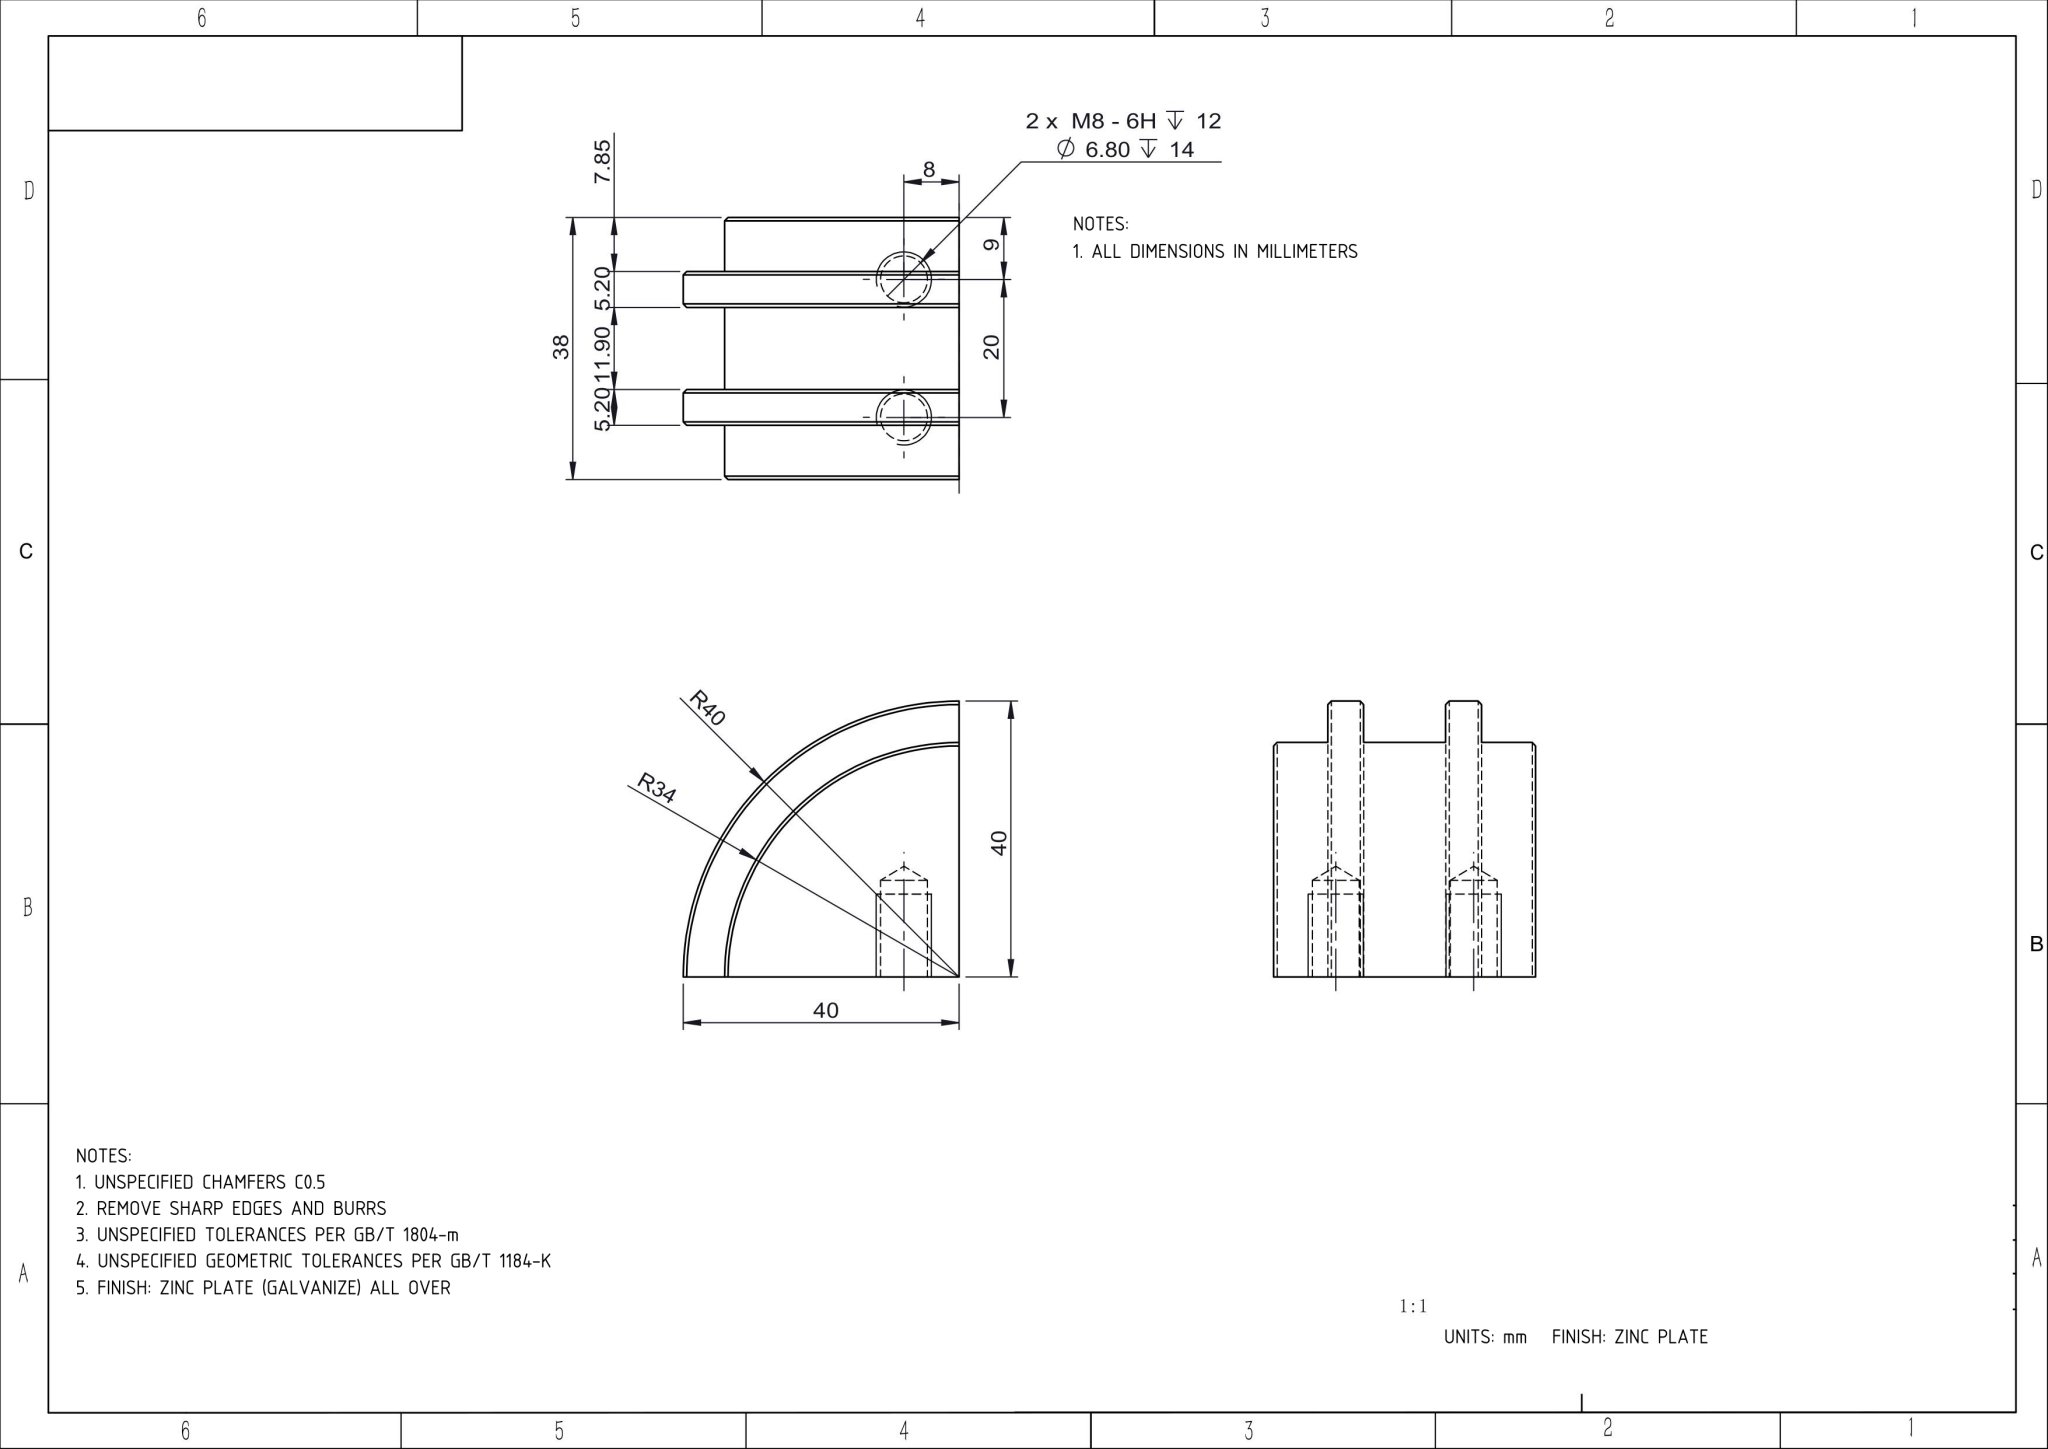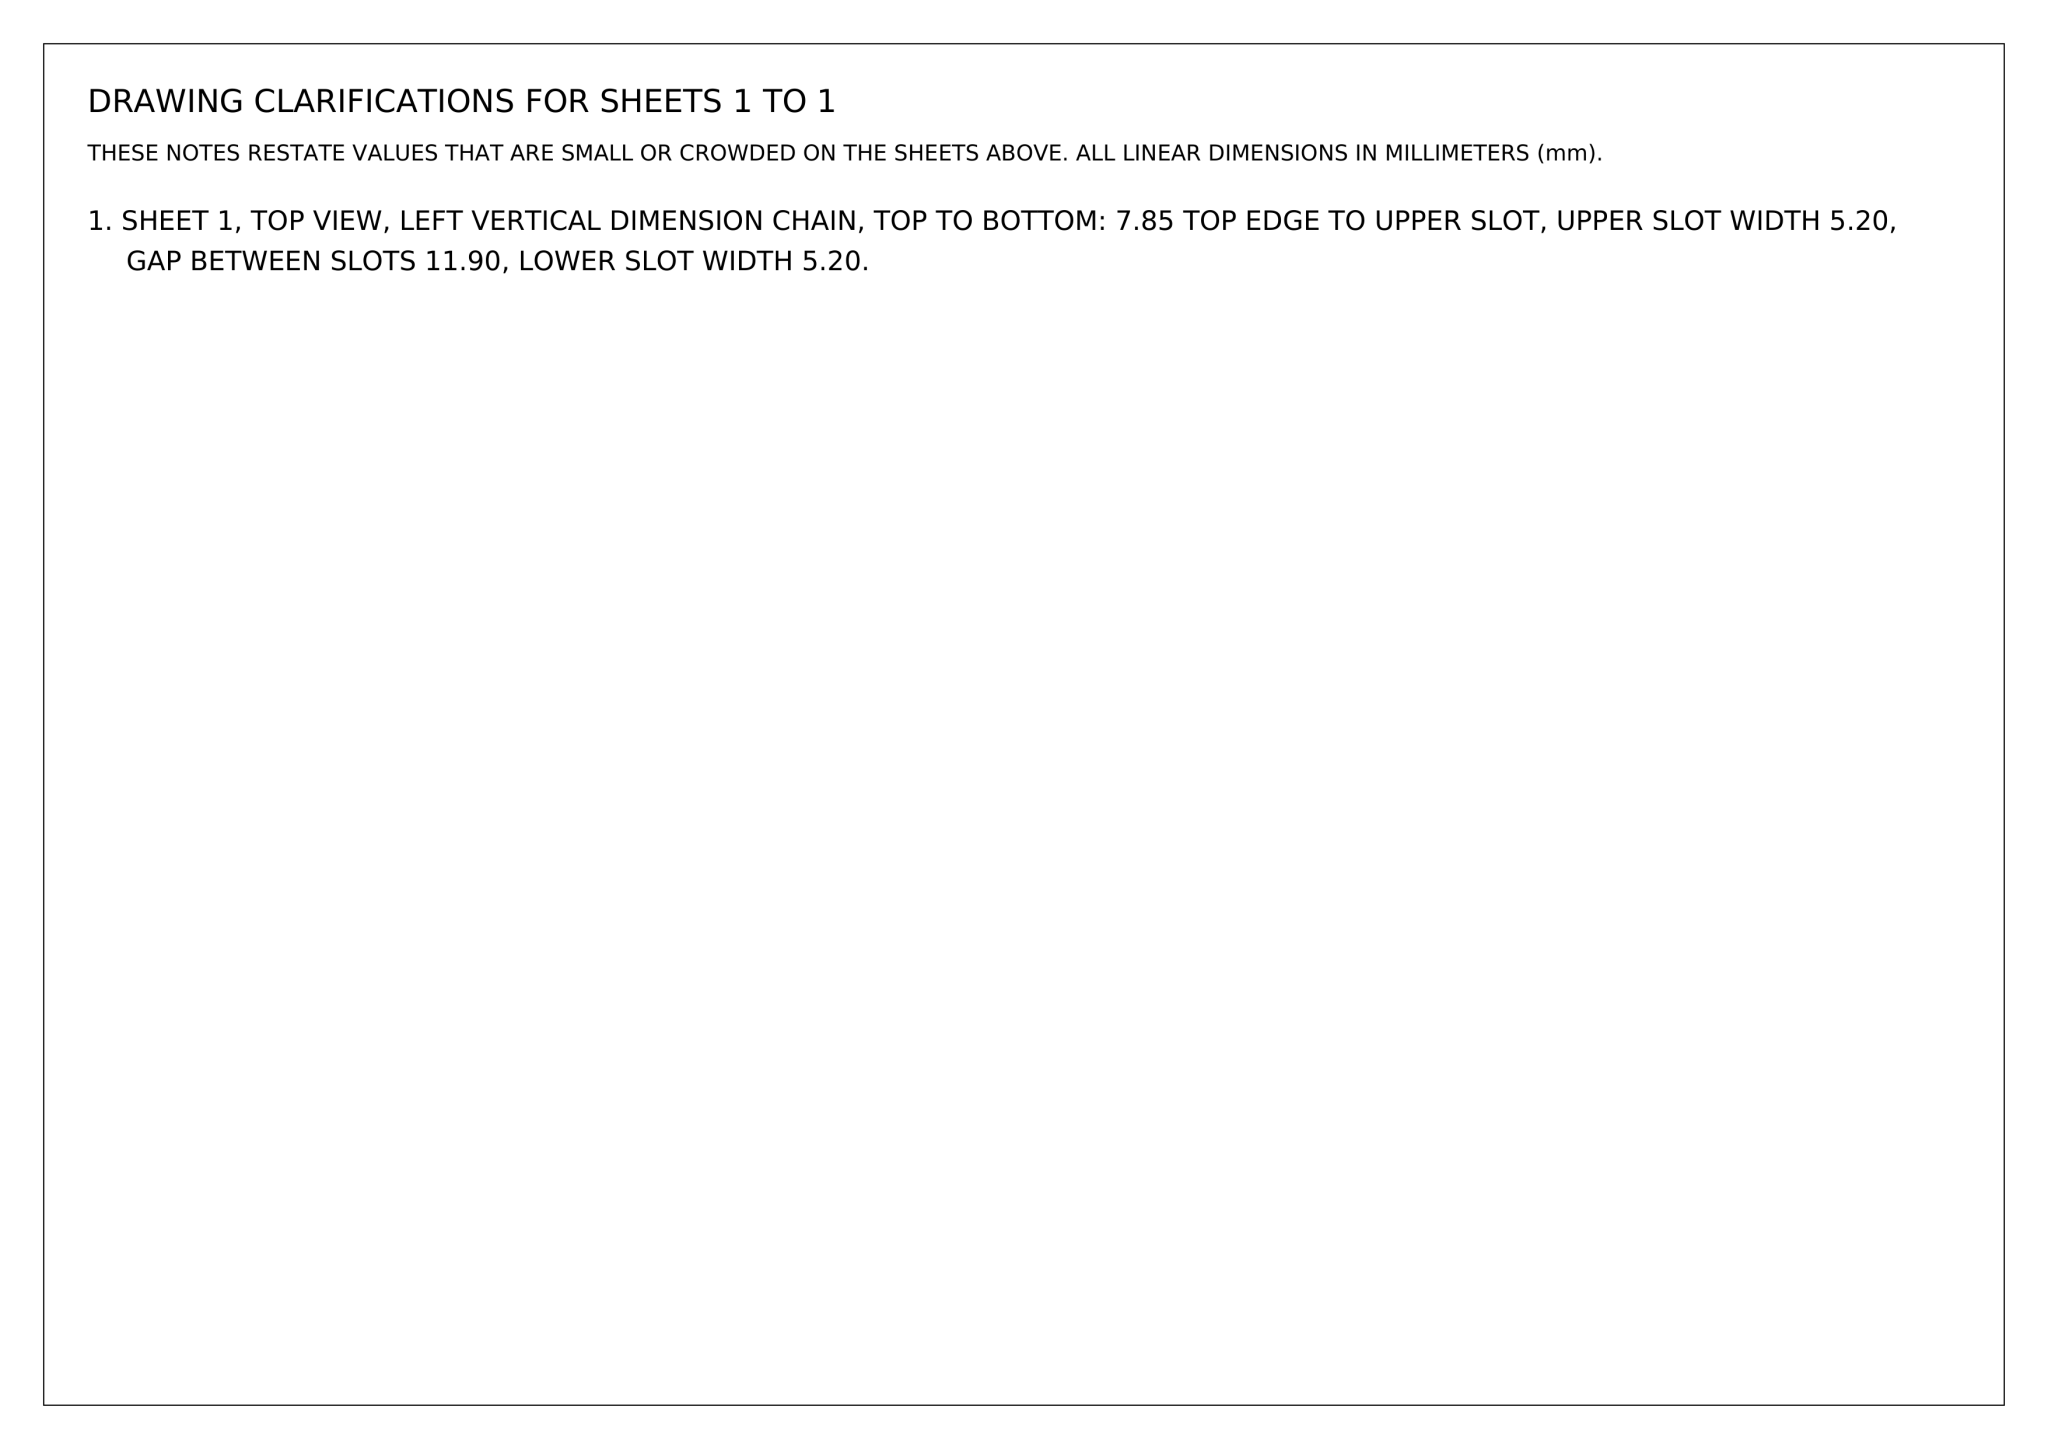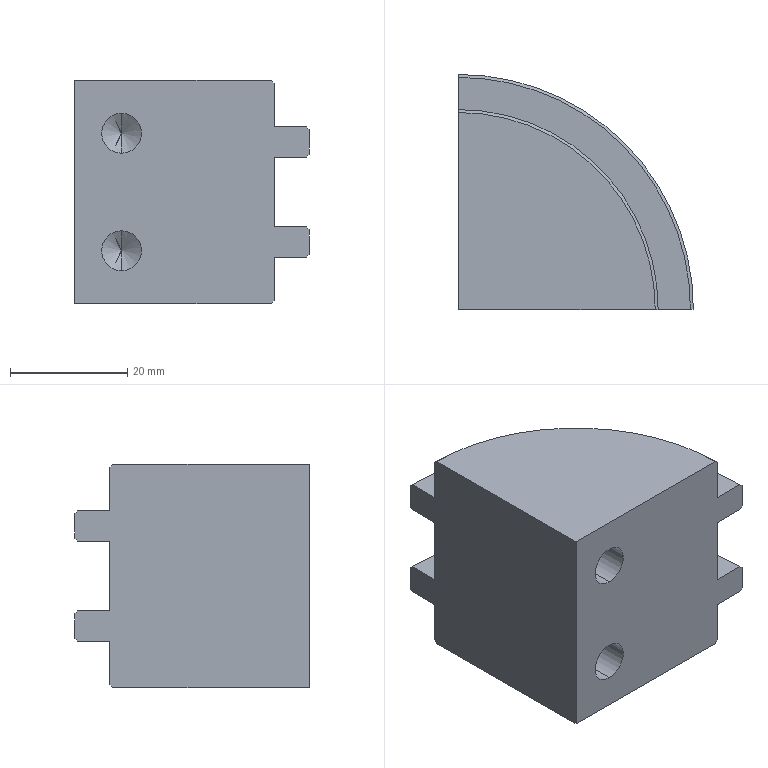Part | NX | mm | 1 solid | 27 faces | box 40 x 40 x 38 mm | volume 37017 mm3 | cone 10 | cylinder 9 | plane 8 | commonest cylinder face diameters 6.8 x4 68 x3 80 x2